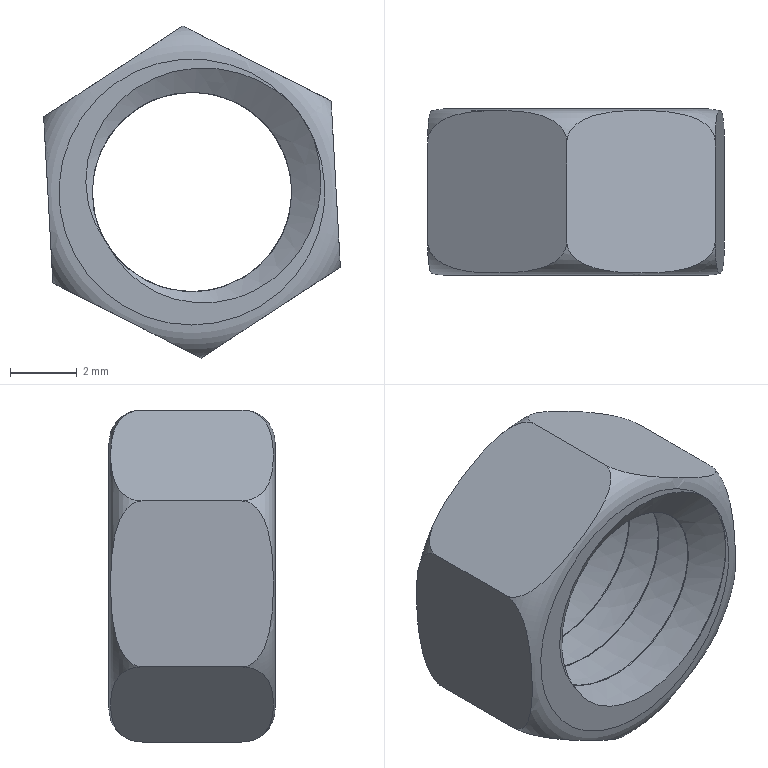Component | NX | JJZ-009_2 | 1 solid | 14 faces | volume 127 mm3 | plane 8 | torus 2 | cylinder 2 | spline 2 | commonest cylinder face diameters 6 x1 8 x1